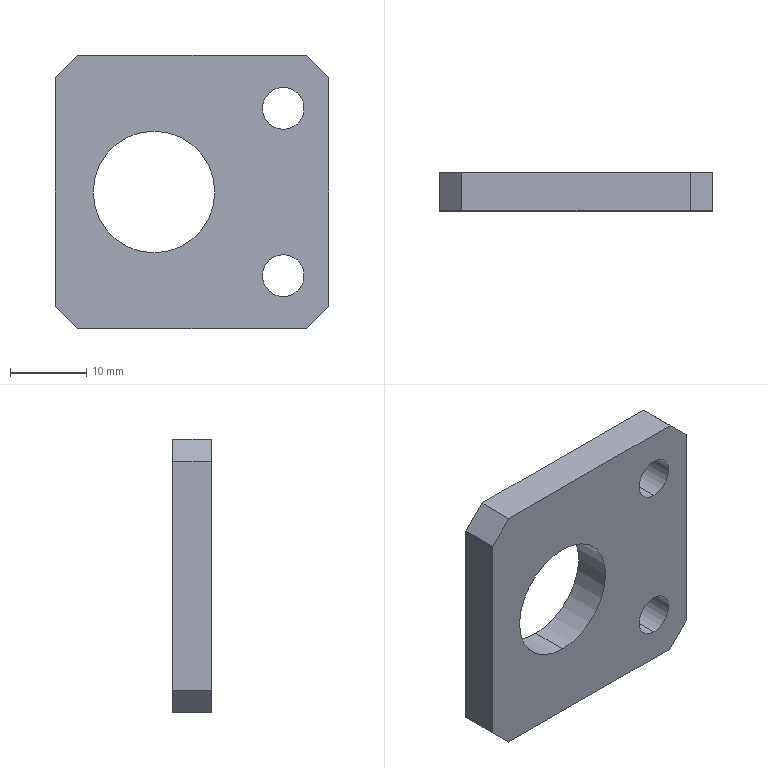Component | SolidWorks | MTCTV2104DJ006-000-0042StopPart-1 | 1 solid | 16 faces | box 36 x 5 x 36 mm | volume 5147 mm3 | plane 10 | cylinder 6 | commonest cylinder face diameters 5.5 x4 16 x2
build123d program:
from build123d import *

# Parameters (mm, degrees)
SKETCH1_W           = 36
SKETCH1_H           = 36
SKETCH1_R           = 8
SKETCH1_R_2         = 2.75
BOSS_EXTRUDE1_DEPTH = 5
CHAMFER1_SIZE       = 3


with BuildPart() as part:
    # Sketch1 → Boss-Extrude1 (new body)
    with BuildSketch(Plane(origin=(0, 0, 0), x_dir=(0, 0, -1), z_dir=(1, 0, 0))):
        Rectangle(SKETCH1_W, SKETCH1_H)
        with Locations((0, 5)):
            Circle(SKETCH1_R, mode=Mode.SUBTRACT)
        with Locations((-11, -12)):
            Circle(SKETCH1_R_2, mode=Mode.SUBTRACT)
        with Locations((11, -12)):
            Circle(SKETCH1_R_2, mode=Mode.SUBTRACT)
    extrude(amount=BOSS_EXTRUDE1_DEPTH)

    # Chamfer1
    chamfer1_edges = [part.edges().sort_by_distance(p)[0] for p in [
        (2.5, -18, -18),
        (2.5, -18, 18),
        (2.5, 18, 18),
        (2.5, 18, -18),
    ]]
    chamfer(chamfer1_edges, length=CHAMFER1_SIZE)


solid = part.part

# Placed as in the assembly
solid = solid.moved(Location((8.798, -105.678, 265.447), (0, 0, 90)))
STEP:
#1=COLOUR_RGB('',0.7922,0.8196,0.9333);
#2=FILL_AREA_STYLE_COLOUR('',#1);
#3=FILL_AREA_STYLE('',(#2));
#4=SURFACE_STYLE_FILL_AREA(#3);
#5=SURFACE_SIDE_STYLE('',(#4));
#6=SURFACE_STYLE_USAGE(.BOTH.,#5);
#7=PRESENTATION_STYLE_ASSIGNMENT((#6));
#8=CARTESIAN_POINT('',(0.8188,-3.964,10.126));
#9=VERTEX_POINT('',#8);
#10=CARTESIAN_POINT('',(0.8188,-3.964,9.909));
#11=VERTEX_POINT('',#10);
#12=CARTESIAN_POINT('',(0.8188,-3.964,10.018));
#13=DIRECTION('',(-0.,1.,-0.));
#14=DIRECTION('',(0.,0.,-1.));
#15=AXIS2_PLACEMENT_3D('',#12,#13,#14);
#16=CIRCLE('',#15,0.1083);
#17=EDGE_CURVE('',#9,#11,#16,.T.);
#18=ORIENTED_EDGE('',*,*,#17,.T.);
#19=CARTESIAN_POINT('',(0.8188,-4.161,9.909));
#20=VERTEX_POINT('',#19);
#21=CARTESIAN_POINT('',(0.8188,-3.964,9.909));
#22=DIRECTION('',(0.,-1.,0.));
#23=VECTOR('',#22,39.37);
#24=LINE('',#21,#23);
#25=EDGE_CURVE('',#11,#20,#24,.T.);
#26=ORIENTED_EDGE('',*,*,#25,.T.);
#27=CARTESIAN_POINT('',(0.8188,-4.161,10.126));
#28=VERTEX_POINT('',#27);
#29=CARTESIAN_POINT('',(0.8188,-4.161,10.018));
#30=DIRECTION('',(-0.,1.,-0.));
#31=DIRECTION('',(0.,0.,-1.));
#32=AXIS2_PLACEMENT_3D('',#29,#30,#31);
#33=CIRCLE('',#32,0.1083);
#34=EDGE_CURVE('',#28,#20,#33,.T.);
#35=ORIENTED_EDGE('',*,*,#34,.F.);
#36=CARTESIAN_POINT('',(0.8188,-3.964,10.126));
#37=DIRECTION('',(0.,-1.,0.));
#38=VECTOR('',#37,39.37);
#39=LINE('',#36,#38);
#40=EDGE_CURVE('',#9,#28,#39,.T.);
#41=ORIENTED_EDGE('',*,*,#40,.F.);
#42=EDGE_LOOP('',(#18,#26,#35,#41));
#43=FACE_OUTER_BOUND('',#42,.T.);
#44=CARTESIAN_POINT('',(0.8188,-3.964,10.018));
#45=DIRECTION('',(0.,-1.,0.));
#46=DIRECTION('',(0.,0.,1.));
#47=AXIS2_PLACEMENT_3D('',#44,#45,#46);
#48=CYLINDRICAL_SURFACE('',#47,0.1083);
#49=ADVANCED_FACE('',(#43),#48,.F.);
#50=CARTESIAN_POINT('',(0.8188,-3.964,10.992));
#51=VERTEX_POINT('',#50);
#52=CARTESIAN_POINT('',(0.8188,-3.964,10.775));
#53=VERTEX_POINT('',#52);
#54=CARTESIAN_POINT('',(0.8188,-3.964,10.884));
#55=DIRECTION('',(-0.,1.,-0.));
#56=DIRECTION('',(0.,0.,-1.));
#57=AXIS2_PLACEMENT_3D('',#54,#55,#56);
#58=CIRCLE('',#57,0.1083);
#59=EDGE_CURVE('',#51,#53,#58,.T.);
#60=ORIENTED_EDGE('',*,*,#59,.T.);
#61=CARTESIAN_POINT('',(0.8188,-4.161,10.775));
#62=VERTEX_POINT('',#61);
#63=CARTESIAN_POINT('',(0.8188,-3.964,10.775));
#64=DIRECTION('',(0.,-1.,0.));
#65=VECTOR('',#64,39.37);
#66=LINE('',#63,#65);
#67=EDGE_CURVE('',#53,#62,#66,.T.);
#68=ORIENTED_EDGE('',*,*,#67,.T.);
#69=CARTESIAN_POINT('',(0.8188,-4.161,10.992));
#70=VERTEX_POINT('',#69);
#71=CARTESIAN_POINT('',(0.8188,-4.161,10.884));
#72=DIRECTION('',(-0.,1.,-0.));
#73=DIRECTION('',(0.,0.,-1.));
#74=AXIS2_PLACEMENT_3D('',#71,#72,#73);
#75=CIRCLE('',#74,0.1083);
#76=EDGE_CURVE('',#70,#62,#75,.T.);
#77=ORIENTED_EDGE('',*,*,#76,.F.);
#78=CARTESIAN_POINT('',(0.8188,-3.964,10.992));
#79=DIRECTION('',(0.,-1.,0.));
#80=VECTOR('',#79,39.37);
#81=LINE('',#78,#80);
#82=EDGE_CURVE('',#51,#70,#81,.T.);
#83=ORIENTED_EDGE('',*,*,#82,.F.);
#84=EDGE_LOOP('',(#60,#68,#77,#83));
#85=FACE_OUTER_BOUND('',#84,.T.);
#86=CARTESIAN_POINT('',(0.8188,-3.964,10.884));
#87=DIRECTION('',(0.,-1.,0.));
#88=DIRECTION('',(0.,0.,1.));
#89=AXIS2_PLACEMENT_3D('',#86,#87,#88);
#90=CYLINDRICAL_SURFACE('',#89,0.1083);
#91=ADVANCED_FACE('',(#85),#90,.F.);
#92=CARTESIAN_POINT('',(0.1495,-3.964,10.766));
#93=VERTEX_POINT('',#92);
#94=CARTESIAN_POINT('',(0.1495,-3.964,10.136));
#95=VERTEX_POINT('',#94);
#96=CARTESIAN_POINT('',(0.1495,-3.964,10.451));
#97=DIRECTION('',(-0.,1.,-0.));
#98=DIRECTION('',(0.,0.,-1.));
#99=AXIS2_PLACEMENT_3D('',#96,#97,#98);
#100=CIRCLE('',#99,0.315);
#101=EDGE_CURVE('',#93,#95,#100,.T.);
#102=ORIENTED_EDGE('',*,*,#101,.T.);
#103=CARTESIAN_POINT('',(0.1495,-4.161,10.136));
#104=VERTEX_POINT('',#103);
#105=CARTESIAN_POINT('',(0.1495,-3.964,10.136));
#106=DIRECTION('',(0.,-1.,0.));
#107=VECTOR('',#106,39.37);
#108=LINE('',#105,#107);
#109=EDGE_CURVE('',#95,#104,#108,.T.);
#110=ORIENTED_EDGE('',*,*,#109,.T.);
#111=CARTESIAN_POINT('',(0.1495,-4.161,10.766));
#112=VERTEX_POINT('',#111);
#113=CARTESIAN_POINT('',(0.1495,-4.161,10.451));
#114=DIRECTION('',(-0.,1.,-0.));
#115=DIRECTION('',(0.,0.,-1.));
#116=AXIS2_PLACEMENT_3D('',#113,#114,#115);
#117=CIRCLE('',#116,0.315);
#118=EDGE_CURVE('',#112,#104,#117,.T.);
#119=ORIENTED_EDGE('',*,*,#118,.F.);
#120=CARTESIAN_POINT('',(0.1495,-3.964,10.766));
#121=DIRECTION('',(0.,-1.,0.));
#122=VECTOR('',#121,39.37);
#123=LINE('',#120,#122);
#124=EDGE_CURVE('',#93,#112,#123,.T.);
#125=ORIENTED_EDGE('',*,*,#124,.F.);
#126=EDGE_LOOP('',(#102,#110,#119,#125));
#127=FACE_OUTER_BOUND('',#126,.T.);
#128=CARTESIAN_POINT('',(0.1495,-3.964,10.451));
#129=DIRECTION('',(0.,-1.,0.));
#130=DIRECTION('',(0.,0.,1.));
#131=AXIS2_PLACEMENT_3D('',#128,#129,#130);
#132=CYLINDRICAL_SURFACE('',#131,0.315);
#133=ADVANCED_FACE('',(#127),#132,.F.);
#134=CARTESIAN_POINT('',(1.055,-3.964,11.041));
#135=VERTEX_POINT('',#134);
#136=CARTESIAN_POINT('',(1.055,-3.964,9.86));
#137=VERTEX_POINT('',#136);
#138=CARTESIAN_POINT('',(1.055,-3.964,11.159));
#139=DIRECTION('',(0.,-0.,-1.));
#140=VECTOR('',#139,39.37);
#141=LINE('',#138,#140);
#142=EDGE_CURVE('',#135,#137,#141,.T.);
#143=ORIENTED_EDGE('',*,*,#142,.T.);
#144=CARTESIAN_POINT('',(0.9369,-3.964,9.742));
#145=VERTEX_POINT('',#144);
#146=CARTESIAN_POINT('',(0.9369,-3.964,9.742));
#147=DIRECTION('',(-0.7071,-0.,-0.7071));
#148=VECTOR('',#147,39.37);
#149=LINE('',#146,#148);
#150=EDGE_CURVE('',#137,#145,#149,.T.);
#151=ORIENTED_EDGE('',*,*,#150,.T.);
#152=CARTESIAN_POINT('',(-0.2442,-3.964,9.742));
#153=VERTEX_POINT('',#152);
#154=CARTESIAN_POINT('',(1.055,-3.964,9.742));
#155=DIRECTION('',(-1.,-0.,-0.));
#156=VECTOR('',#155,39.37);
#157=LINE('',#154,#156);
#158=EDGE_CURVE('',#145,#153,#157,.T.);
#159=ORIENTED_EDGE('',*,*,#158,.T.);
#160=CARTESIAN_POINT('',(-0.3623,-3.964,9.86));
#161=VERTEX_POINT('',#160);
#162=CARTESIAN_POINT('',(-0.3623,-3.964,9.86));
#163=DIRECTION('',(-0.7071,0.,0.7071));
#164=VECTOR('',#163,39.37);
#165=LINE('',#162,#164);
#166=EDGE_CURVE('',#153,#161,#165,.T.);
#167=ORIENTED_EDGE('',*,*,#166,.T.);
#168=CARTESIAN_POINT('',(-0.3623,-3.964,11.041));
#169=VERTEX_POINT('',#168);
#170=CARTESIAN_POINT('',(-0.3623,-3.964,11.159));
#171=DIRECTION('',(-0.,0.,1.));
#172=VECTOR('',#171,39.37);
#173=LINE('',#170,#172);
#174=EDGE_CURVE('',#161,#169,#173,.T.);
#175=ORIENTED_EDGE('',*,*,#174,.T.);
#176=CARTESIAN_POINT('',(-0.2442,-3.964,11.159));
#177=VERTEX_POINT('',#176);
#178=CARTESIAN_POINT('',(-0.2442,-3.964,11.159));
#179=DIRECTION('',(0.7071,0.,0.7071));
#180=VECTOR('',#179,39.37);
#181=LINE('',#178,#180);
#182=EDGE_CURVE('',#169,#177,#181,.T.);
#183=ORIENTED_EDGE('',*,*,#182,.T.);
#184=CARTESIAN_POINT('',(0.9369,-3.964,11.159));
#185=VERTEX_POINT('',#184);
#186=CARTESIAN_POINT('',(1.055,-3.964,11.159));
#187=DIRECTION('',(1.,0.,0.));
#188=VECTOR('',#187,39.37);
#189=LINE('',#186,#188);
#190=EDGE_CURVE('',#177,#185,#189,.T.);
#191=ORIENTED_EDGE('',*,*,#190,.T.);
#192=CARTESIAN_POINT('',(1.055,-3.964,11.041));
#193=DIRECTION('',(0.7071,-0.,-0.7071));
#194=VECTOR('',#193,39.37);
#195=LINE('',#192,#194);
#196=EDGE_CURVE('',#185,#135,#195,.T.);
#197=ORIENTED_EDGE('',*,*,#196,.T.);
#198=EDGE_LOOP('',(#143,#151,#159,#167,#175,#183,#191,#197));
#199=FACE_OUTER_BOUND('',#198,.T.);
#200=ORIENTED_EDGE('',*,*,#101,.F.);
#201=CARTESIAN_POINT('',(0.1495,-3.964,10.451));
#202=DIRECTION('',(-0.,1.,-0.));
#203=DIRECTION('',(0.,0.,-1.));
#204=AXIS2_PLACEMENT_3D('',#201,#202,#203);
#205=CIRCLE('',#204,0.315);
#206=EDGE_CURVE('',#95,#93,#205,.T.);
#207=ORIENTED_EDGE('',*,*,#206,.F.);
#208=EDGE_LOOP('',(#200,#207));
#209=FACE_BOUND('',#208,.T.);
#210=ORIENTED_EDGE('',*,*,#59,.F.);
#211=CARTESIAN_POINT('',(0.8188,-3.964,10.884));
#212=DIRECTION('',(-0.,1.,-0.));
#213=DIRECTION('',(0.,0.,-1.));
#214=AXIS2_PLACEMENT_3D('',#211,#212,#213);
#215=CIRCLE('',#214,0.1083);
#216=EDGE_CURVE('',#53,#51,#215,.T.);
#217=ORIENTED_EDGE('',*,*,#216,.F.);
#218=EDGE_LOOP('',(#210,#217));
#219=FACE_BOUND('',#218,.T.);
#220=ORIENTED_EDGE('',*,*,#17,.F.);
#221=CARTESIAN_POINT('',(0.8188,-3.964,10.018));
#222=DIRECTION('',(-0.,1.,-0.));
#223=DIRECTION('',(0.,0.,-1.));
#224=AXIS2_PLACEMENT_3D('',#221,#222,#223);
#225=CIRCLE('',#224,0.1083);
#226=EDGE_CURVE('',#11,#9,#225,.T.);
#227=ORIENTED_EDGE('',*,*,#226,.F.);
#228=EDGE_LOOP('',(#220,#227));
#229=FACE_BOUND('',#228,.T.);
#230=CARTESIAN_POINT('',(0.3464,-3.964,10.451));
#231=DIRECTION('',(0.,-1.,0.));
#232=DIRECTION('',(-0.,0.,1.));
#233=AXIS2_PLACEMENT_3D('',#230,#231,#232);
#234=PLANE('',#233);
#235=ADVANCED_FACE('',(#199,#209,#219,#229),#234,.F.);
#236=ORIENTED_EDGE('',*,*,#76,.T.);
#237=CARTESIAN_POINT('',(0.8188,-4.161,10.884));
#238=DIRECTION('',(-0.,1.,-0.));
#239=DIRECTION('',(0.,0.,-1.));
#240=AXIS2_PLACEMENT_3D('',#237,#238,#239);
#241=CIRCLE('',#240,0.1083);
#242=EDGE_CURVE('',#62,#70,#241,.T.);
#243=ORIENTED_EDGE('',*,*,#242,.T.);
#244=EDGE_LOOP('',(#236,#243));
#245=FACE_BOUND('',#244,.T.);
#246=CARTESIAN_POINT('',(0.9369,-4.161,9.742));
#247=VERTEX_POINT('',#246);
#248=CARTESIAN_POINT('',(-0.2442,-4.161,9.742));
#249=VERTEX_POINT('',#248);
#250=CARTESIAN_POINT('',(1.055,-4.161,9.742));
#251=DIRECTION('',(-1.,-0.,-0.));
#252=VECTOR('',#251,39.37);
#253=LINE('',#250,#252);
#254=EDGE_CURVE('',#247,#249,#253,.T.);
#255=ORIENTED_EDGE('',*,*,#254,.F.);
#256=CARTESIAN_POINT('',(1.055,-4.161,9.86));
#257=VERTEX_POINT('',#256);
#258=CARTESIAN_POINT('',(0.996,-4.161,9.801));
#259=DIRECTION('',(0.7071,0.,0.7071));
#260=VECTOR('',#259,39.37);
#261=LINE('',#258,#260);
#262=EDGE_CURVE('',#247,#257,#261,.T.);
#263=ORIENTED_EDGE('',*,*,#262,.T.);
#264=CARTESIAN_POINT('',(1.055,-4.161,11.041));
#265=VERTEX_POINT('',#264);
#266=CARTESIAN_POINT('',(1.055,-4.161,11.159));
#267=DIRECTION('',(0.,-0.,-1.));
#268=VECTOR('',#267,39.37);
#269=LINE('',#266,#268);
#270=EDGE_CURVE('',#265,#257,#269,.T.);
#271=ORIENTED_EDGE('',*,*,#270,.F.);
#272=CARTESIAN_POINT('',(0.9369,-4.161,11.159));
#273=VERTEX_POINT('',#272);
#274=CARTESIAN_POINT('',(0.996,-4.161,11.1));
#275=DIRECTION('',(-0.7071,0.,0.7071));
#276=VECTOR('',#275,39.37);
#277=LINE('',#274,#276);
#278=EDGE_CURVE('',#265,#273,#277,.T.);
#279=ORIENTED_EDGE('',*,*,#278,.T.);
#280=CARTESIAN_POINT('',(-0.2442,-4.161,11.159));
#281=VERTEX_POINT('',#280);
#282=CARTESIAN_POINT('',(1.055,-4.161,11.159));
#283=DIRECTION('',(1.,0.,0.));
#284=VECTOR('',#283,39.37);
#285=LINE('',#282,#284);
#286=EDGE_CURVE('',#281,#273,#285,.T.);
#287=ORIENTED_EDGE('',*,*,#286,.F.);
#288=CARTESIAN_POINT('',(-0.3623,-4.161,11.041));
#289=VERTEX_POINT('',#288);
#290=CARTESIAN_POINT('',(-0.3032,-4.161,11.1));
#291=DIRECTION('',(-0.7071,-0.,-0.7071));
#292=VECTOR('',#291,39.37);
#293=LINE('',#290,#292);
#294=EDGE_CURVE('',#281,#289,#293,.T.);
#295=ORIENTED_EDGE('',*,*,#294,.T.);
#296=CARTESIAN_POINT('',(-0.3623,-4.161,9.86));
#297=VERTEX_POINT('',#296);
#298=CARTESIAN_POINT('',(-0.3623,-4.161,11.159));
#299=DIRECTION('',(-0.,0.,1.));
#300=VECTOR('',#299,39.37);
#301=LINE('',#298,#300);
#302=EDGE_CURVE('',#297,#289,#301,.T.);
#303=ORIENTED_EDGE('',*,*,#302,.F.);
#304=CARTESIAN_POINT('',(-0.3032,-4.161,9.801));
#305=DIRECTION('',(0.7071,-0.,-0.7071));
#306=VECTOR('',#305,39.37);
#307=LINE('',#304,#306);
#308=EDGE_CURVE('',#297,#249,#307,.T.);
#309=ORIENTED_EDGE('',*,*,#308,.T.);
#310=EDGE_LOOP('',(#255,#263,#271,#279,#287,#295,#303,#309));
#311=FACE_OUTER_BOUND('',#310,.T.);
#312=ORIENTED_EDGE('',*,*,#118,.T.);
#313=CARTESIAN_POINT('',(0.1495,-4.161,10.451));
#314=DIRECTION('',(-0.,1.,-0.));
#315=DIRECTION('',(0.,0.,-1.));
#316=AXIS2_PLACEMENT_3D('',#313,#314,#315);
#317=CIRCLE('',#316,0.315);
#318=EDGE_CURVE('',#104,#112,#317,.T.);
#319=ORIENTED_EDGE('',*,*,#318,.T.);
#320=EDGE_LOOP('',(#312,#319));
#321=FACE_BOUND('',#320,.T.);
#322=ORIENTED_EDGE('',*,*,#34,.T.);
#323=CARTESIAN_POINT('',(0.8188,-4.161,10.018));
#324=DIRECTION('',(-0.,1.,-0.));
#325=DIRECTION('',(0.,0.,-1.));
#326=AXIS2_PLACEMENT_3D('',#323,#324,#325);
#327=CIRCLE('',#326,0.1083);
#328=EDGE_CURVE('',#20,#28,#327,.T.);
#329=ORIENTED_EDGE('',*,*,#328,.T.);
#330=EDGE_LOOP('',(#322,#329));
#331=FACE_BOUND('',#330,.T.);
#332=CARTESIAN_POINT('',(0.3464,-4.161,10.451));
#333=DIRECTION('',(0.,-1.,0.));
#334=DIRECTION('',(-0.,0.,1.));
#335=AXIS2_PLACEMENT_3D('',#332,#333,#334);
#336=PLANE('',#335);
#337=ADVANCED_FACE('',(#245,#311,#321,#331),#336,.T.);
#338=ORIENTED_EDGE('',*,*,#158,.F.);
#339=CARTESIAN_POINT('',(0.9369,-3.964,9.742));
#340=DIRECTION('',(0.,-1.,0.));
#341=VECTOR('',#340,39.37);
#342=LINE('',#339,#341);
#343=EDGE_CURVE('',#145,#247,#342,.T.);
#344=ORIENTED_EDGE('',*,*,#343,.T.);
#345=ORIENTED_EDGE('',*,*,#254,.T.);
#346=CARTESIAN_POINT('',(-0.2442,-3.964,9.742));
#347=DIRECTION('',(-0.,1.,-0.));
#348=VECTOR('',#347,39.37);
#349=LINE('',#346,#348);
#350=EDGE_CURVE('',#249,#153,#349,.T.);
#351=ORIENTED_EDGE('',*,*,#350,.T.);
#352=EDGE_LOOP('',(#338,#344,#345,#351));
#353=FACE_OUTER_BOUND('',#352,.T.);
#354=CARTESIAN_POINT('',(1.055,-3.964,9.742));
#355=DIRECTION('',(-0.,0.,1.));
#356=DIRECTION('',(-0.,1.,-0.));
#357=AXIS2_PLACEMENT_3D('',#354,#355,#356);
#358=PLANE('',#357);
#359=ADVANCED_FACE('',(#353),#358,.F.);
#360=ORIENTED_EDGE('',*,*,#174,.F.);
#361=CARTESIAN_POINT('',(-0.3623,-3.964,9.86));
#362=DIRECTION('',(0.,-1.,0.));
#363=VECTOR('',#362,39.37);
#364=LINE('',#361,#363);
#365=EDGE_CURVE('',#161,#297,#364,.T.);
#366=ORIENTED_EDGE('',*,*,#365,.T.);
#367=ORIENTED_EDGE('',*,*,#302,.T.);
#368=CARTESIAN_POINT('',(-0.3623,-3.964,11.041));
#369=DIRECTION('',(-0.,1.,-0.));
#370=VECTOR('',#369,39.37);
#371=LINE('',#368,#370);
#372=EDGE_CURVE('',#289,#169,#371,.T.);
#373=ORIENTED_EDGE('',*,*,#372,.T.);
#374=EDGE_LOOP('',(#360,#366,#367,#373));
#375=FACE_OUTER_BOUND('',#374,.T.);
#376=CARTESIAN_POINT('',(-0.3623,-3.964,11.159));
#377=DIRECTION('',(1.,0.,0.));
#378=DIRECTION('',(0.,-0.,-1.));
#379=AXIS2_PLACEMENT_3D('',#376,#377,#378);
#380=PLANE('',#379);
#381=ADVANCED_FACE('',(#375),#380,.F.);
#382=ORIENTED_EDGE('',*,*,#286,.T.);
#383=CARTESIAN_POINT('',(0.9369,-3.964,11.159));
#384=DIRECTION('',(-0.,1.,-0.));
#385=VECTOR('',#384,39.37);
#386=LINE('',#383,#385);
#387=EDGE_CURVE('',#273,#185,#386,.T.);
#388=ORIENTED_EDGE('',*,*,#387,.T.);
#389=ORIENTED_EDGE('',*,*,#190,.F.);
#390=CARTESIAN_POINT('',(-0.2442,-3.964,11.159));
#391=DIRECTION('',(0.,-1.,0.));
#392=VECTOR('',#391,39.37);
#393=LINE('',#390,#392);
#394=EDGE_CURVE('',#177,#281,#393,.T.);
#395=ORIENTED_EDGE('',*,*,#394,.T.);
#396=EDGE_LOOP('',(#382,#388,#389,#395));
#397=FACE_OUTER_BOUND('',#396,.T.);
#398=CARTESIAN_POINT('',(1.055,-3.964,11.159));
#399=DIRECTION('',(0.,-0.,-1.));
#400=DIRECTION('',(0.,-1.,0.));
#401=AXIS2_PLACEMENT_3D('',#398,#399,#400);
#402=PLANE('',#401);
#403=ADVANCED_FACE('',(#397),#402,.F.);
#404=ORIENTED_EDGE('',*,*,#270,.T.);
#405=CARTESIAN_POINT('',(1.055,-3.964,9.86));
#406=DIRECTION('',(-0.,1.,-0.));
#407=VECTOR('',#406,39.37);
#408=LINE('',#405,#407);
#409=EDGE_CURVE('',#257,#137,#408,.T.);
#410=ORIENTED_EDGE('',*,*,#409,.T.);
#411=ORIENTED_EDGE('',*,*,#142,.F.);
#412=CARTESIAN_POINT('',(1.055,-3.964,11.041));
#413=DIRECTION('',(0.,-1.,0.));
#414=VECTOR('',#413,39.37);
#415=LINE('',#412,#414);
#416=EDGE_CURVE('',#135,#265,#415,.T.);
#417=ORIENTED_EDGE('',*,*,#416,.T.);
#418=EDGE_LOOP('',(#404,#410,#411,#417));
#419=FACE_OUTER_BOUND('',#418,.T.);
#420=CARTESIAN_POINT('',(1.055,-3.964,11.159));
#421=DIRECTION('',(-1.,-0.,-0.));
#422=DIRECTION('',(-0.,0.,1.));
#423=AXIS2_PLACEMENT_3D('',#420,#421,#422);
#424=PLANE('',#423);
#425=ADVANCED_FACE('',(#419),#424,.F.);
#426=ORIENTED_EDGE('',*,*,#109,.F.);
#427=ORIENTED_EDGE('',*,*,#206,.T.);
#428=ORIENTED_EDGE('',*,*,#124,.T.);
#429=ORIENTED_EDGE('',*,*,#318,.F.);
#430=EDGE_LOOP('',(#426,#427,#428,#429));
#431=FACE_OUTER_BOUND('',#430,.T.);
#432=CARTESIAN_POINT('',(0.1495,-3.964,10.451));
#433=DIRECTION('',(0.,-1.,0.));
#434=DIRECTION('',(0.,0.,1.));
#435=AXIS2_PLACEMENT_3D('',#432,#433,#434);
#436=CYLINDRICAL_SURFACE('',#435,0.315);
#437=ADVANCED_FACE('',(#431),#436,.F.);
#438=ORIENTED_EDGE('',*,*,#67,.F.);
#439=ORIENTED_EDGE('',*,*,#216,.T.);
#440=ORIENTED_EDGE('',*,*,#82,.T.);
#441=ORIENTED_EDGE('',*,*,#242,.F.);
#442=EDGE_LOOP('',(#438,#439,#440,#441));
#443=FACE_OUTER_BOUND('',#442,.T.);
#444=CARTESIAN_POINT('',(0.8188,-3.964,10.884));
#445=DIRECTION('',(0.,-1.,0.));
#446=DIRECTION('',(0.,0.,1.));
#447=AXIS2_PLACEMENT_3D('',#444,#445,#446);
#448=CYLINDRICAL_SURFACE('',#447,0.1083);
#449=ADVANCED_FACE('',(#443),#448,.F.);
#450=ORIENTED_EDGE('',*,*,#25,.F.);
#451=ORIENTED_EDGE('',*,*,#226,.T.);
#452=ORIENTED_EDGE('',*,*,#40,.T.);
#453=ORIENTED_EDGE('',*,*,#328,.F.);
#454=EDGE_LOOP('',(#450,#451,#452,#453));
#455=FACE_OUTER_BOUND('',#454,.T.);
#456=CARTESIAN_POINT('',(0.8188,-3.964,10.018));
#457=DIRECTION('',(0.,-1.,0.));
#458=DIRECTION('',(0.,0.,1.));
#459=AXIS2_PLACEMENT_3D('',#456,#457,#458);
#460=CYLINDRICAL_SURFACE('',#459,0.1083);
#461=ADVANCED_FACE('',(#455),#460,.F.);
#462=ORIENTED_EDGE('',*,*,#150,.F.);
#463=ORIENTED_EDGE('',*,*,#409,.F.);
#464=ORIENTED_EDGE('',*,*,#262,.F.);
#465=ORIENTED_EDGE('',*,*,#343,.F.);
#466=EDGE_LOOP('',(#462,#463,#464,#465));
#467=FACE_OUTER_BOUND('',#466,.T.);
#468=CARTESIAN_POINT('',(0.9369,-3.964,9.742));
#469=DIRECTION('',(-0.7071,0.,0.7071));
#470=DIRECTION('',(0.,-1.,0.));
#471=AXIS2_PLACEMENT_3D('',#468,#469,#470);
#472=PLANE('',#471);
#473=ADVANCED_FACE('',(#467),#472,.F.);
#474=ORIENTED_EDGE('',*,*,#196,.F.);
#475=ORIENTED_EDGE('',*,*,#387,.F.);
#476=ORIENTED_EDGE('',*,*,#278,.F.);
#477=ORIENTED_EDGE('',*,*,#416,.F.);
#478=EDGE_LOOP('',(#474,#475,#476,#477));
#479=FACE_OUTER_BOUND('',#478,.T.);
#480=CARTESIAN_POINT('',(1.055,-3.964,11.041));
#481=DIRECTION('',(-0.7071,-0.,-0.7071));
#482=DIRECTION('',(0.,-1.,0.));
#483=AXIS2_PLACEMENT_3D('',#480,#481,#482);
#484=PLANE('',#483);
#485=ADVANCED_FACE('',(#479),#484,.F.);
#486=ORIENTED_EDGE('',*,*,#166,.F.);
#487=ORIENTED_EDGE('',*,*,#350,.F.);
#488=ORIENTED_EDGE('',*,*,#308,.F.);
#489=ORIENTED_EDGE('',*,*,#365,.F.);
#490=EDGE_LOOP('',(#486,#487,#488,#489));
#491=FACE_OUTER_BOUND('',#490,.T.);
#492=CARTESIAN_POINT('',(-0.3623,-3.964,9.86));
#493=DIRECTION('',(0.7071,0.,0.7071));
#494=DIRECTION('',(0.,-1.,0.));
#495=AXIS2_PLACEMENT_3D('',#492,#493,#494);
#496=PLANE('',#495);
#497=ADVANCED_FACE('',(#491),#496,.F.);
#498=ORIENTED_EDGE('',*,*,#182,.F.);
#499=ORIENTED_EDGE('',*,*,#372,.F.);
#500=ORIENTED_EDGE('',*,*,#294,.F.);
#501=ORIENTED_EDGE('',*,*,#394,.F.);
#502=EDGE_LOOP('',(#498,#499,#500,#501));
#503=FACE_OUTER_BOUND('',#502,.T.);
#504=CARTESIAN_POINT('',(-0.2442,-3.964,11.159));
#505=DIRECTION('',(0.7071,-0.,-0.7071));
#506=DIRECTION('',(0.,-1.,0.));
#507=AXIS2_PLACEMENT_3D('',#504,#505,#506);
#508=PLANE('',#507);
#509=ADVANCED_FACE('',(#503),#508,.F.);
#510=CLOSED_SHELL('',(#49,#91,#133,#235,#337,#359,#381,#403,#425,#437,#449,#461,#473,#485,#497,#509));
#511=MANIFOLD_SOLID_BREP('',#510);
#512=STYLED_ITEM('',(#7),#511);
#513=(LENGTH_UNIT()NAMED_UNIT(*)SI_UNIT($,.METRE.));
#514=LENGTH_MEASURE_WITH_UNIT(LENGTH_MEASURE(0.0254),#513);
#515=DIMENSIONAL_EXPONENTS(1.,0.,0.,0.,0.,0.,0.);
#516=(CONVERSION_BASED_UNIT('',#514)LENGTH_UNIT()NAMED_UNIT(#515));
#517=UNCERTAINTY_MEASURE_WITH_UNIT(LENGTH_MEASURE(0.00001),#516,'','');
#518=(NAMED_UNIT(*)PLANE_ANGLE_UNIT()SI_UNIT($,.RADIAN.));
#519=(NAMED_UNIT(*)SI_UNIT($,.STERADIAN.)SOLID_ANGLE_UNIT());
#520=(GEOMETRIC_REPRESENTATION_CONTEXT(3)GLOBAL_UNCERTAINTY_ASSIGNED_CONTEXT((#517))GLOBAL_UNIT_ASSIGNED_CONTEXT((#516,#518,#519))REPRESENTATION_CONTEXT('',''));
#521=MECHANICAL_DESIGN_GEOMETRIC_PRESENTATION_REPRESENTATION('',(#512),#520);
#522=CARTESIAN_POINT('',(0.,0.,0.));
#523=DIRECTION('',(0.,0.,1.));
#524=DIRECTION('',(1.,0.,0.));
#525=AXIS2_PLACEMENT_3D('',#522,#523,#524);
#526=(LENGTH_UNIT()NAMED_UNIT(*)SI_UNIT($,.METRE.));
#527=LENGTH_MEASURE_WITH_UNIT(LENGTH_MEASURE(0.0254),#526);
#528=DIMENSIONAL_EXPONENTS(1.,0.,0.,0.,0.,0.,0.);
#529=(CONVERSION_BASED_UNIT('',#527)LENGTH_UNIT()NAMED_UNIT(#528));
#530=UNCERTAINTY_MEASURE_WITH_UNIT(LENGTH_MEASURE(0.00001),#529,'','');
#531=(NAMED_UNIT(*)PLANE_ANGLE_UNIT()SI_UNIT($,.RADIAN.));
#532=(NAMED_UNIT(*)SI_UNIT($,.STERADIAN.)SOLID_ANGLE_UNIT());
#533=(GEOMETRIC_REPRESENTATION_CONTEXT(3)GLOBAL_UNCERTAINTY_ASSIGNED_CONTEXT((#530))GLOBAL_UNIT_ASSIGNED_CONTEXT((#529,#531,#532))REPRESENTATION_CONTEXT('',''));
#534=ADVANCED_BREP_SHAPE_REPRESENTATION('',(#511,#525),#533);
#535=PRESENTATION_LAYER_ASSIGNMENT('','',(#512));